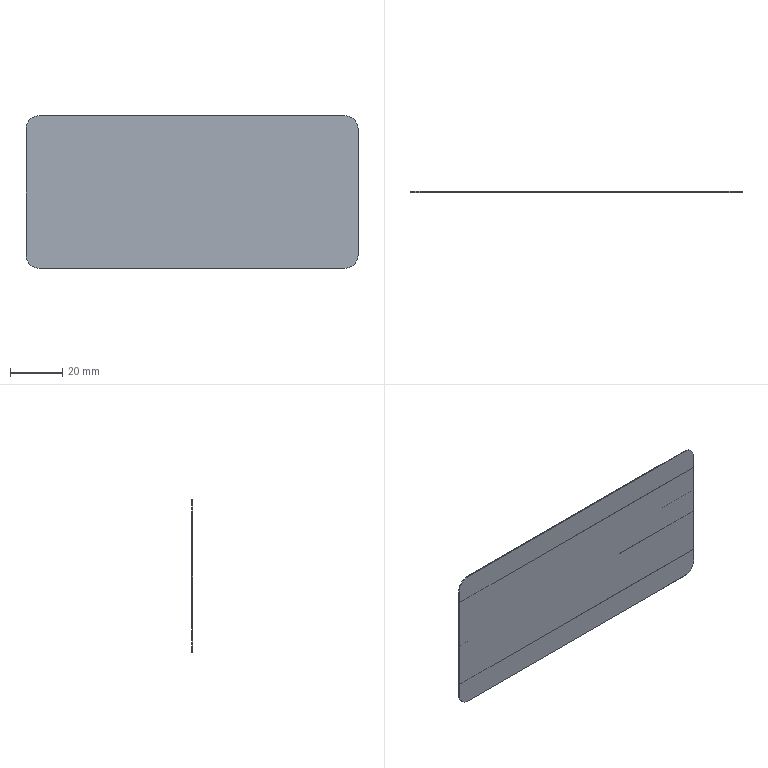Component | SolidWorks | OuterBagStorageAssembly-1_PackagingBagLength-1 | 1 solid | 20 faces | box 127.5 x 0.45 x 58.5 mm | volume 1591 mm3 | plane 16 | cylinder 4 | commonest cylinder face diameters 10 x4
build123d program:
from build123d import *

# Parameters (mm, degrees)
SKETCH1_W           = 58.5
SKETCH1_H           = 127.5
BOSS_EXTRUDE1_DEPTH = 0.0375
SKETCH2_W           = 10
SKETCH2_H           = 127.5
BOSS_EXTRUDE2_DEPTH = 0.15
SKETCH3_W           = 58.5
SKETCH3_H           = 127.5
BOSS_EXTRUDE3_DEPTH = 0.075
SKETCH4_W           = 10
SKETCH4_H           = 127.5
BOSS_EXTRUDE4_DEPTH = 0.15
SKETCH5_W           = 9.925
SKETCH5_H           = 0.075
CUT_EXTRUDE1_DEPTH  = 131.813
FILLET1_R           = 5


with BuildPart() as part:
    # Sketch1 → Boss-Extrude1 (new, symmetric)
    with BuildSketch(Plane(origin=(0, 0, 0), x_dir=(1, 0, 0), z_dir=(0, 1, 0))):
        Rectangle(SKETCH1_W, SKETCH1_H)
    extrude(amount=BOSS_EXTRUDE1_DEPTH, both=True)

    # Sketch2 → Boss-Extrude2 (add)
    with BuildSketch(Plane(origin=(0, 0.0375, 0), x_dir=(1, 0, 0), z_dir=(0, 1, 0))):
        with Locations((-24.25, 0)):
            Rectangle(SKETCH2_W, SKETCH2_H)
        with Locations((24.25, 0)):
            Rectangle(SKETCH2_W, SKETCH2_H)
    extrude(amount=BOSS_EXTRUDE2_DEPTH)

    # Sketch3 → Boss-Extrude3 (add)
    with BuildSketch(Plane(origin=(0, 0.1875, 0), x_dir=(1, 0, 0), z_dir=(0, 1, 0))):
        Rectangle(SKETCH3_W, SKETCH3_H)
    extrude(amount=BOSS_EXTRUDE3_DEPTH)

    # Sketch4 → Boss-Extrude4 (add)
    with BuildSketch(Plane(origin=(0, 0.2625, 0), x_dir=(1, 0, 0), z_dir=(0, 1, 0))):
        with Locations((-3.75, 0)):
            Rectangle(SKETCH4_W, SKETCH4_H)
    extrude(amount=BOSS_EXTRUDE4_DEPTH)

    # Sketch5 → Cut-Extrude1 (cut, through all)
    with BuildSketch(Plane.XY.offset(63.75)):
        with Locations((-3.788, 0.3)):
            Rectangle(SKETCH5_W, SKETCH5_H)
    extrude(amount=-CUT_EXTRUDE1_DEPTH, mode=Mode.SUBTRACT)

    # Fillet1
    fillet1_edges = [part.edges().sort_by_distance(p)[0] for p in [
        (29.25, 0.1125, 63.75),
        (-29.25, 0.1125, 63.75),
        (29.25, 0.1125, -63.75),
        (-29.25, 0.1125, -63.75),
    ]]
    fillet(fillet1_edges, radius=FILLET1_R)


solid = part.part

# Placed as in the assembly
solid = solid.moved(Location((-314.796, 159.368, 374.168), (0, 90, 0)))